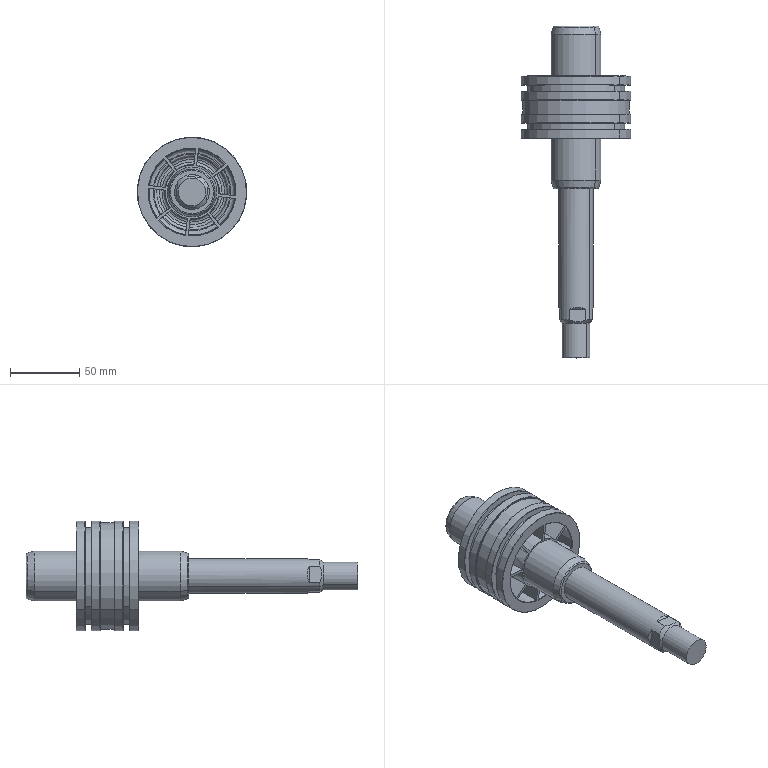Component | SolidWorks | SC-80x75(000)-1_2-1 | 1 solid | 252 faces | volume 236233 mm3 | plane 84 | spline 74 | cone 72 | cylinder 22 | commonest cylinder face diameters 79 x8 36 x4 70 x4 25 x2 20 x2 76.9 x2